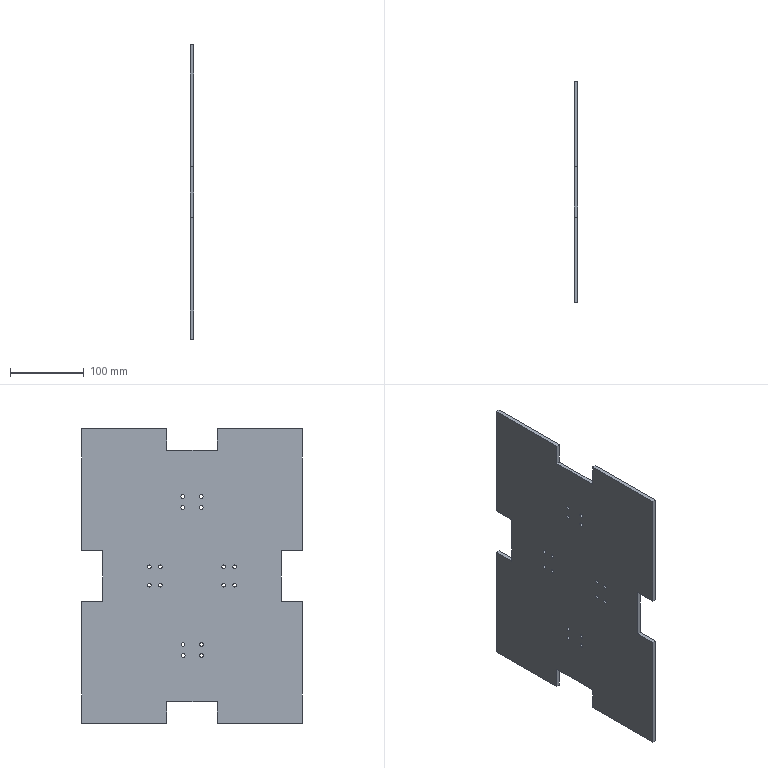Component | SolidWorks | Chassis-1 | 1 solid | 54 faces | box 5 x 300 x 400 mm | volume 558402 mm3 | cylinder 32 | plane 22 | commonest cylinder face diameters 5 x28 5.034 x2 5.135 x2
build123d program:
from build123d import *

# Parameters (mm, degrees)
SKETCH1_W           = 400
SKETCH1_H           = 300
BOSS_EXTRUDE1_DEPTH = 5
SKETCH2_R           = 2.5
SKETCH2_R_2         = 2.568
SKETCH2_R_3         = 2.517
SKETCH2_W           = 39.202
SKETCH2_H           = 69
SKETCH2_W_2         = 69
SKETCH2_H_2         = 109.927
SKETCH2_W_3         = 55.808
SKETCH2_H_3         = 94.104
CUT_EXTRUDE1_DEPTH  = 10


with BuildPart() as part:
    # Sketch1 → Boss-Extrude1 (new body)
    with BuildSketch(Plane.XY):
        Rectangle(SKETCH1_W, SKETCH1_H)
    extrude(amount=BOSS_EXTRUDE1_DEPTH)

    # Sketch2 → Cut-Extrude1 (cut)
    with BuildSketch(Plane(origin=(0, 0, 0), x_dir=(-1, 0, 0), z_dir=(0, 0, -1))):
        with Locations((-93, 12.032)):
            Circle(SKETCH2_R)
        with Locations((-93, -12.968)):
            Circle(SKETCH2_R)
        with Locations((-108, -12.968)):
            Circle(SKETCH2_R)
        with Locations((-108, 12.032)):
            Circle(SKETCH2_R_2)
        with Locations((-12.5, -43)):
            Circle(SKETCH2_R)
        with Locations((-12.5, -58)):
            Circle(SKETCH2_R)
        with Locations((12.5, -58)):
            Circle(SKETCH2_R)
        with Locations((12.5, -43)):
            Circle(SKETCH2_R)
        with Locations((93, -12.5)):
            Circle(SKETCH2_R)
        with Locations((93, 12.5)):
            Circle(SKETCH2_R)
        with Locations((108, 12.5)):
            Circle(SKETCH2_R)
        with Locations((-12.5, 58)):
            Circle(SKETCH2_R)
        with Locations((-12.5, 43)):
            Circle(SKETCH2_R)
        with Locations((12.5, 43)):
            Circle(SKETCH2_R_3)
        with Locations((12.5, 58)):
            Circle(SKETCH2_R)
        with Locations((108, -12.5)):
            Circle(SKETCH2_R)
        with Locations((190.601, 0)):
            Rectangle(SKETCH2_W, SKETCH2_H)
        with Locations((0, -175.964)):
            Rectangle(SKETCH2_W_2, SKETCH2_H_2)
        with Locations((-198.904, 0)):
            Rectangle(SKETCH2_W_3, SKETCH2_H)
        with Locations((0, 168.052)):
            Rectangle(SKETCH2_W_2, SKETCH2_H_3)
    extrude(amount=-CUT_EXTRUDE1_DEPTH, mode=Mode.SUBTRACT)


solid = part.part

# Placed as in the assembly
solid = solid.moved(Location((-320, 0, -542.97), (0, 90, 0)))